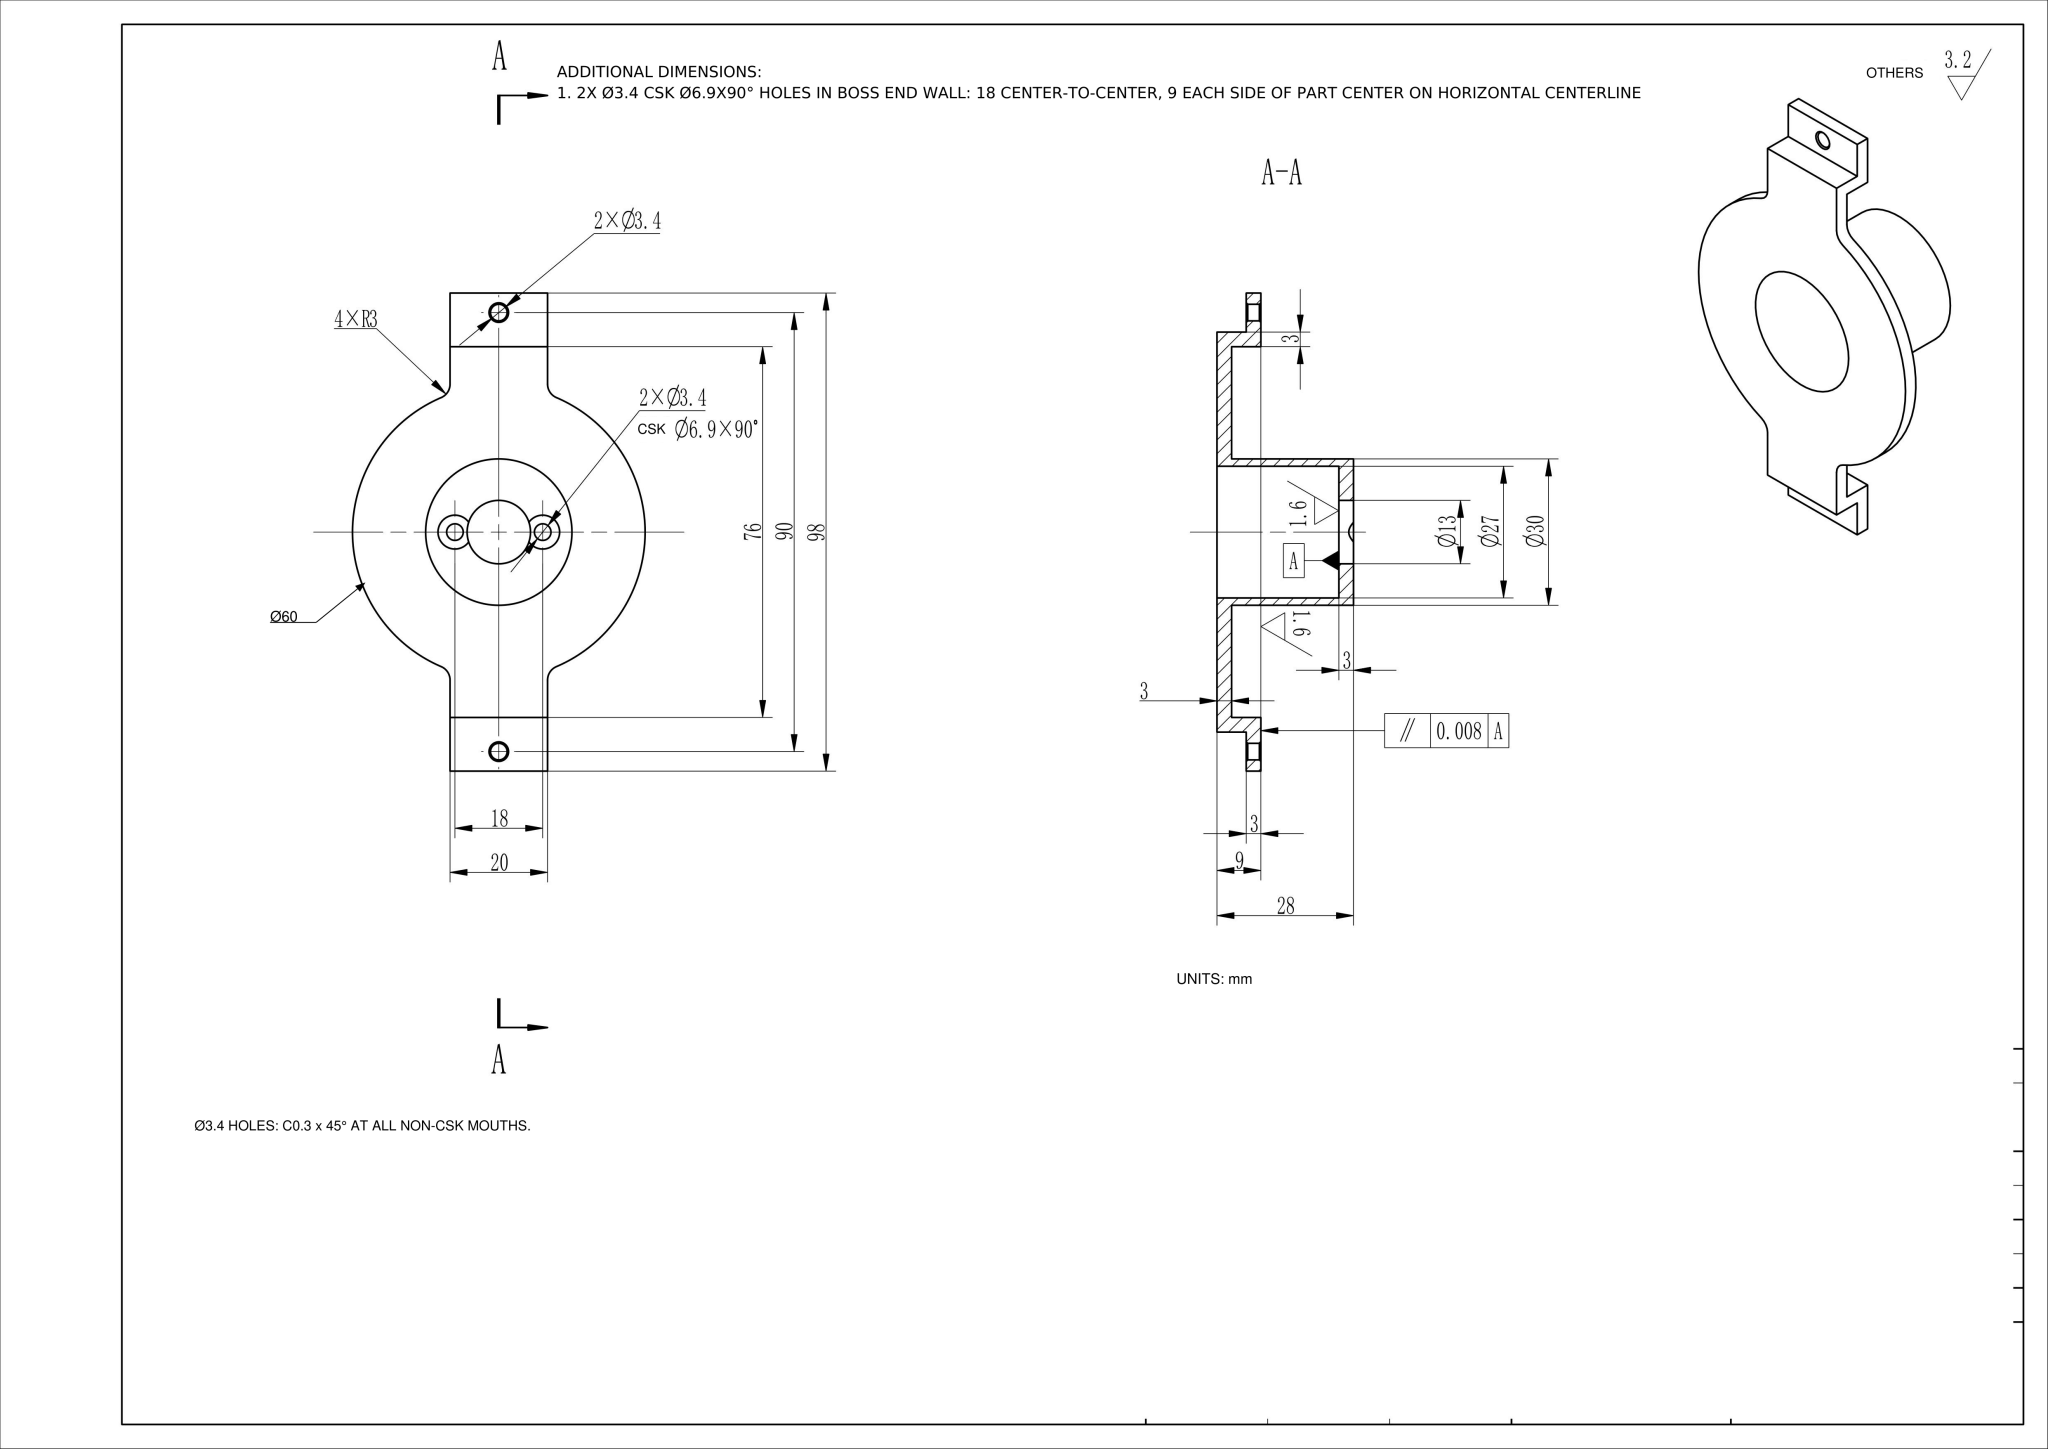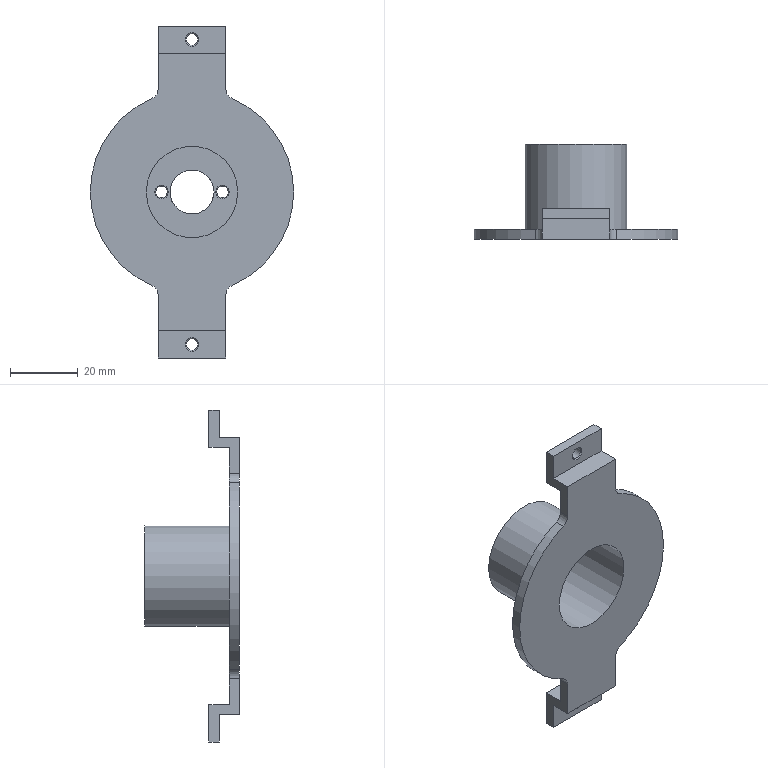Part | NX | mm | 1 solid | 39 faces | box 60 x 28 x 98 mm | volume 14363 mm3 | plane 18 | cylinder 13 | cone 8 | commonest cylinder face diameters 3.4 x4 6 x4 60 x2 30 x1 13 x1 27 x1